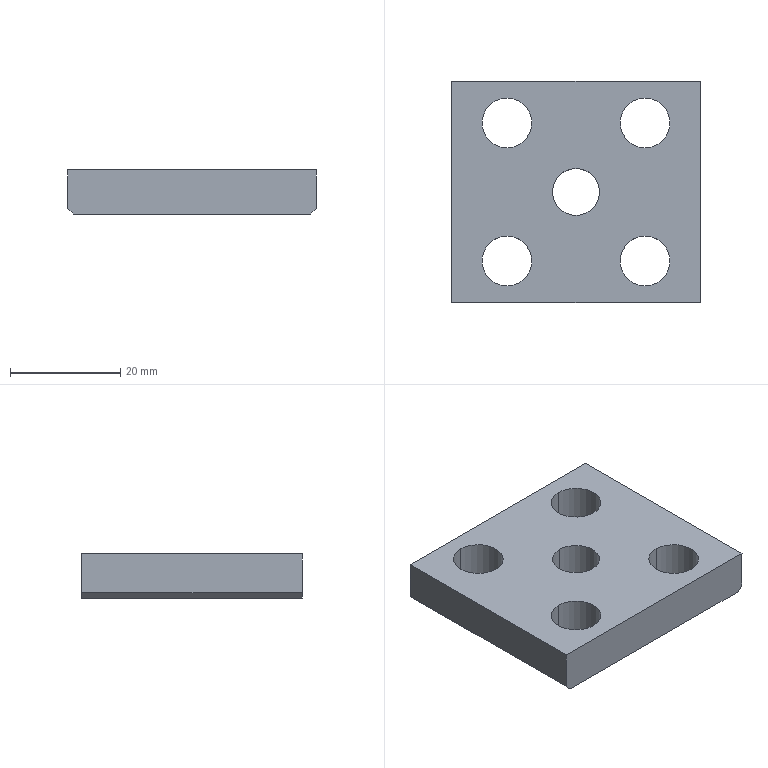Component | SolidWorks | Frame-1_PressurePlate-1 | 1 solid | 18 faces | box 45 x 40 x 8 mm | volume 11870 mm3 | cylinder 10 | plane 8 | commonest cylinder face diameters 9 x8 8.5 x2 | material Plain Carbon Steel
STEP:
#1=CARTESIAN_POINT('',(-171.122,344.501,294.147));
#2=VERTEX_POINT('',#1);
#3=CARTESIAN_POINT('',(-171.122,344.835,294.147));
#4=VERTEX_POINT('',#3);
#5=CARTESIAN_POINT('',(-171.122,344.668,294.147));
#6=DIRECTION('',(-0.,0.,-1.));
#7=DIRECTION('',(0.,1.,0.));
#8=AXIS2_PLACEMENT_3D('',#5,#6,#7);
#9=CIRCLE('',#8,0.1673);
#10=EDGE_CURVE('',#2,#4,#9,.T.);
#11=ORIENTED_EDGE('',*,*,#10,.F.);
#12=CARTESIAN_POINT('',(-171.122,344.501,293.832));
#13=VERTEX_POINT('',#12);
#14=CARTESIAN_POINT('',(-171.122,344.501,293.832));
#15=DIRECTION('',(-0.,0.,-1.));
#16=VECTOR('',#15,39.37);
#17=LINE('',#14,#16);
#18=EDGE_CURVE('',#2,#13,#17,.T.);
#19=ORIENTED_EDGE('',*,*,#18,.T.);
#20=CARTESIAN_POINT('',(-171.122,344.835,293.832));
#21=VERTEX_POINT('',#20);
#22=CARTESIAN_POINT('',(-171.122,344.668,293.832));
#23=DIRECTION('',(-0.,0.,-1.));
#24=DIRECTION('',(0.,1.,0.));
#25=AXIS2_PLACEMENT_3D('',#22,#23,#24);
#26=CIRCLE('',#25,0.1673);
#27=EDGE_CURVE('',#13,#21,#26,.T.);
#28=ORIENTED_EDGE('',*,*,#27,.T.);
#29=CARTESIAN_POINT('',(-171.122,344.835,293.832));
#30=DIRECTION('',(-0.,0.,-1.));
#31=VECTOR('',#30,39.37);
#32=LINE('',#29,#31);
#33=EDGE_CURVE('',#4,#21,#32,.T.);
#34=ORIENTED_EDGE('',*,*,#33,.F.);
#35=EDGE_LOOP('',(#11,#19,#28,#34));
#36=FACE_OUTER_BOUND('',#35,.T.);
#37=CARTESIAN_POINT('',(-171.122,344.668,293.832));
#38=DIRECTION('',(-0.,0.,-1.));
#39=DIRECTION('',(0.,1.,0.));
#40=AXIS2_PLACEMENT_3D('',#37,#38,#39);
#41=CYLINDRICAL_SURFACE('',#40,0.1673);
#42=ADVANCED_FACE('',(#36),#41,.F.);
#43=CARTESIAN_POINT('',(-171.614,343.999,293.832));
#44=VERTEX_POINT('',#43);
#45=CARTESIAN_POINT('',(-171.614,344.353,293.832));
#46=VERTEX_POINT('',#45);
#47=CARTESIAN_POINT('',(-171.614,344.176,293.832));
#48=DIRECTION('',(-0.,0.,-1.));
#49=DIRECTION('',(0.,1.,0.));
#50=AXIS2_PLACEMENT_3D('',#47,#48,#49);
#51=CIRCLE('',#50,0.1772);
#52=EDGE_CURVE('',#44,#46,#51,.T.);
#53=ORIENTED_EDGE('',*,*,#52,.T.);
#54=CARTESIAN_POINT('',(-171.614,344.353,294.147));
#55=VERTEX_POINT('',#54);
#56=CARTESIAN_POINT('',(-171.614,344.353,293.832));
#57=DIRECTION('',(0.,-0.,1.));
#58=VECTOR('',#57,39.37);
#59=LINE('',#56,#58);
#60=EDGE_CURVE('',#46,#55,#59,.T.);
#61=ORIENTED_EDGE('',*,*,#60,.T.);
#62=CARTESIAN_POINT('',(-171.614,343.999,294.147));
#63=VERTEX_POINT('',#62);
#64=CARTESIAN_POINT('',(-171.614,344.176,294.147));
#65=DIRECTION('',(-0.,0.,-1.));
#66=DIRECTION('',(0.,1.,0.));
#67=AXIS2_PLACEMENT_3D('',#64,#65,#66);
#68=CIRCLE('',#67,0.1772);
#69=EDGE_CURVE('',#63,#55,#68,.T.);
#70=ORIENTED_EDGE('',*,*,#69,.F.);
#71=CARTESIAN_POINT('',(-171.614,343.999,293.832));
#72=DIRECTION('',(0.,-0.,1.));
#73=VECTOR('',#72,39.37);
#74=LINE('',#71,#73);
#75=EDGE_CURVE('',#44,#63,#74,.T.);
#76=ORIENTED_EDGE('',*,*,#75,.F.);
#77=EDGE_LOOP('',(#53,#61,#70,#76));
#78=FACE_OUTER_BOUND('',#77,.T.);
#79=CARTESIAN_POINT('',(-171.614,344.176,293.832));
#80=DIRECTION('',(0.,-0.,1.));
#81=DIRECTION('',(-0.,-1.,0.));
#82=AXIS2_PLACEMENT_3D('',#79,#80,#81);
#83=CYLINDRICAL_SURFACE('',#82,0.1772);
#84=ADVANCED_FACE('',(#78),#83,.F.);
#85=CARTESIAN_POINT('',(-171.614,344.983,293.832));
#86=VERTEX_POINT('',#85);
#87=CARTESIAN_POINT('',(-171.614,345.337,293.832));
#88=VERTEX_POINT('',#87);
#89=CARTESIAN_POINT('',(-171.614,345.16,293.832));
#90=DIRECTION('',(-0.,0.,-1.));
#91=DIRECTION('',(0.,1.,0.));
#92=AXIS2_PLACEMENT_3D('',#89,#90,#91);
#93=CIRCLE('',#92,0.1772);
#94=EDGE_CURVE('',#86,#88,#93,.T.);
#95=ORIENTED_EDGE('',*,*,#94,.T.);
#96=CARTESIAN_POINT('',(-171.614,345.337,294.147));
#97=VERTEX_POINT('',#96);
#98=CARTESIAN_POINT('',(-171.614,345.337,293.832));
#99=DIRECTION('',(0.,-0.,1.));
#100=VECTOR('',#99,39.37);
#101=LINE('',#98,#100);
#102=EDGE_CURVE('',#88,#97,#101,.T.);
#103=ORIENTED_EDGE('',*,*,#102,.T.);
#104=CARTESIAN_POINT('',(-171.614,344.983,294.147));
#105=VERTEX_POINT('',#104);
#106=CARTESIAN_POINT('',(-171.614,345.16,294.147));
#107=DIRECTION('',(-0.,0.,-1.));
#108=DIRECTION('',(0.,1.,0.));
#109=AXIS2_PLACEMENT_3D('',#106,#107,#108);
#110=CIRCLE('',#109,0.1772);
#111=EDGE_CURVE('',#105,#97,#110,.T.);
#112=ORIENTED_EDGE('',*,*,#111,.F.);
#113=CARTESIAN_POINT('',(-171.614,344.983,293.832));
#114=DIRECTION('',(0.,-0.,1.));
#115=VECTOR('',#114,39.37);
#116=LINE('',#113,#115);
#117=EDGE_CURVE('',#86,#105,#116,.T.);
#118=ORIENTED_EDGE('',*,*,#117,.F.);
#119=EDGE_LOOP('',(#95,#103,#112,#118));
#120=FACE_OUTER_BOUND('',#119,.T.);
#121=CARTESIAN_POINT('',(-171.614,345.16,293.832));
#122=DIRECTION('',(0.,-0.,1.));
#123=DIRECTION('',(-0.,-1.,0.));
#124=AXIS2_PLACEMENT_3D('',#121,#122,#123);
#125=CYLINDRICAL_SURFACE('',#124,0.1772);
#126=ADVANCED_FACE('',(#120),#125,.F.);
#127=CARTESIAN_POINT('',(-170.63,343.999,293.832));
#128=VERTEX_POINT('',#127);
#129=CARTESIAN_POINT('',(-170.63,344.353,293.832));
#130=VERTEX_POINT('',#129);
#131=CARTESIAN_POINT('',(-170.63,344.176,293.832));
#132=DIRECTION('',(-0.,0.,-1.));
#133=DIRECTION('',(0.,1.,0.));
#134=AXIS2_PLACEMENT_3D('',#131,#132,#133);
#135=CIRCLE('',#134,0.1772);
#136=EDGE_CURVE('',#128,#130,#135,.T.);
#137=ORIENTED_EDGE('',*,*,#136,.T.);
#138=CARTESIAN_POINT('',(-170.63,344.353,294.147));
#139=VERTEX_POINT('',#138);
#140=CARTESIAN_POINT('',(-170.63,344.353,293.832));
#141=DIRECTION('',(0.,-0.,1.));
#142=VECTOR('',#141,39.37);
#143=LINE('',#140,#142);
#144=EDGE_CURVE('',#130,#139,#143,.T.);
#145=ORIENTED_EDGE('',*,*,#144,.T.);
#146=CARTESIAN_POINT('',(-170.63,343.999,294.147));
#147=VERTEX_POINT('',#146);
#148=CARTESIAN_POINT('',(-170.63,344.176,294.147));
#149=DIRECTION('',(-0.,0.,-1.));
#150=DIRECTION('',(0.,1.,0.));
#151=AXIS2_PLACEMENT_3D('',#148,#149,#150);
#152=CIRCLE('',#151,0.1772);
#153=EDGE_CURVE('',#147,#139,#152,.T.);
#154=ORIENTED_EDGE('',*,*,#153,.F.);
#155=CARTESIAN_POINT('',(-170.63,343.999,293.832));
#156=DIRECTION('',(0.,-0.,1.));
#157=VECTOR('',#156,39.37);
#158=LINE('',#155,#157);
#159=EDGE_CURVE('',#128,#147,#158,.T.);
#160=ORIENTED_EDGE('',*,*,#159,.F.);
#161=EDGE_LOOP('',(#137,#145,#154,#160));
#162=FACE_OUTER_BOUND('',#161,.T.);
#163=CARTESIAN_POINT('',(-170.63,344.176,293.832));
#164=DIRECTION('',(0.,-0.,1.));
#165=DIRECTION('',(-0.,-1.,0.));
#166=AXIS2_PLACEMENT_3D('',#163,#164,#165);
#167=CYLINDRICAL_SURFACE('',#166,0.1772);
#168=ADVANCED_FACE('',(#162),#167,.F.);
#169=CARTESIAN_POINT('',(-170.63,344.983,293.832));
#170=VERTEX_POINT('',#169);
#171=CARTESIAN_POINT('',(-170.63,345.337,293.832));
#172=VERTEX_POINT('',#171);
#173=CARTESIAN_POINT('',(-170.63,345.16,293.832));
#174=DIRECTION('',(-0.,0.,-1.));
#175=DIRECTION('',(0.,1.,0.));
#176=AXIS2_PLACEMENT_3D('',#173,#174,#175);
#177=CIRCLE('',#176,0.1772);
#178=EDGE_CURVE('',#170,#172,#177,.T.);
#179=ORIENTED_EDGE('',*,*,#178,.T.);
#180=CARTESIAN_POINT('',(-170.63,345.337,294.147));
#181=VERTEX_POINT('',#180);
#182=CARTESIAN_POINT('',(-170.63,345.337,293.832));
#183=DIRECTION('',(0.,-0.,1.));
#184=VECTOR('',#183,39.37);
#185=LINE('',#182,#184);
#186=EDGE_CURVE('',#172,#181,#185,.T.);
#187=ORIENTED_EDGE('',*,*,#186,.T.);
#188=CARTESIAN_POINT('',(-170.63,344.983,294.147));
#189=VERTEX_POINT('',#188);
#190=CARTESIAN_POINT('',(-170.63,345.16,294.147));
#191=DIRECTION('',(-0.,0.,-1.));
#192=DIRECTION('',(0.,1.,0.));
#193=AXIS2_PLACEMENT_3D('',#190,#191,#192);
#194=CIRCLE('',#193,0.1772);
#195=EDGE_CURVE('',#189,#181,#194,.T.);
#196=ORIENTED_EDGE('',*,*,#195,.F.);
#197=CARTESIAN_POINT('',(-170.63,344.983,293.832));
#198=DIRECTION('',(0.,-0.,1.));
#199=VECTOR('',#198,39.37);
#200=LINE('',#197,#199);
#201=EDGE_CURVE('',#170,#189,#200,.T.);
#202=ORIENTED_EDGE('',*,*,#201,.F.);
#203=EDGE_LOOP('',(#179,#187,#196,#202));
#204=FACE_OUTER_BOUND('',#203,.T.);
#205=CARTESIAN_POINT('',(-170.63,345.16,293.832));
#206=DIRECTION('',(0.,-0.,1.));
#207=DIRECTION('',(-0.,-1.,0.));
#208=AXIS2_PLACEMENT_3D('',#205,#206,#207);
#209=CYLINDRICAL_SURFACE('',#208,0.1772);
#210=ADVANCED_FACE('',(#204),#209,.F.);
#211=CARTESIAN_POINT('',(-171.122,344.668,293.832));
#212=DIRECTION('',(-0.,0.,-1.));
#213=DIRECTION('',(0.,1.,0.));
#214=AXIS2_PLACEMENT_3D('',#211,#212,#213);
#215=CIRCLE('',#214,0.1673);
#216=EDGE_CURVE('',#21,#13,#215,.T.);
#217=ORIENTED_EDGE('',*,*,#216,.F.);
#218=ORIENTED_EDGE('',*,*,#27,.F.);
#219=EDGE_LOOP('',(#217,#218));
#220=FACE_BOUND('',#219,.T.);
#221=CARTESIAN_POINT('',(-170.276,343.88,293.832));
#222=VERTEX_POINT('',#221);
#223=CARTESIAN_POINT('',(-171.969,343.88,293.832));
#224=VERTEX_POINT('',#223);
#225=CARTESIAN_POINT('',(-172.008,343.88,293.832));
#226=DIRECTION('',(-1.,0.,0.));
#227=VECTOR('',#226,39.37);
#228=LINE('',#225,#227);
#229=EDGE_CURVE('',#222,#224,#228,.T.);
#230=ORIENTED_EDGE('',*,*,#229,.T.);
#231=CARTESIAN_POINT('',(-171.969,345.455,293.832));
#232=VERTEX_POINT('',#231);
#233=CARTESIAN_POINT('',(-171.969,343.88,293.832));
#234=DIRECTION('',(0.,1.,0.));
#235=VECTOR('',#234,39.37);
#236=LINE('',#233,#235);
#237=EDGE_CURVE('',#224,#232,#236,.T.);
#238=ORIENTED_EDGE('',*,*,#237,.T.);
#239=CARTESIAN_POINT('',(-170.276,345.455,293.832));
#240=VERTEX_POINT('',#239);
#241=CARTESIAN_POINT('',(-172.008,345.455,293.832));
#242=DIRECTION('',(1.,-0.,-0.));
#243=VECTOR('',#242,39.37);
#244=LINE('',#241,#243);
#245=EDGE_CURVE('',#232,#240,#244,.T.);
#246=ORIENTED_EDGE('',*,*,#245,.T.);
#247=CARTESIAN_POINT('',(-170.276,343.88,293.832));
#248=DIRECTION('',(-0.,-1.,-0.));
#249=VECTOR('',#248,39.37);
#250=LINE('',#247,#249);
#251=EDGE_CURVE('',#240,#222,#250,.T.);
#252=ORIENTED_EDGE('',*,*,#251,.T.);
#253=EDGE_LOOP('',(#230,#238,#246,#252));
#254=FACE_OUTER_BOUND('',#253,.T.);
#255=ORIENTED_EDGE('',*,*,#178,.F.);
#256=CARTESIAN_POINT('',(-170.63,345.16,293.832));
#257=DIRECTION('',(-0.,0.,-1.));
#258=DIRECTION('',(0.,1.,0.));
#259=AXIS2_PLACEMENT_3D('',#256,#257,#258);
#260=CIRCLE('',#259,0.1772);
#261=EDGE_CURVE('',#172,#170,#260,.T.);
#262=ORIENTED_EDGE('',*,*,#261,.F.);
#263=EDGE_LOOP('',(#255,#262));
#264=FACE_BOUND('',#263,.T.);
#265=ORIENTED_EDGE('',*,*,#136,.F.);
#266=CARTESIAN_POINT('',(-170.63,344.176,293.832));
#267=DIRECTION('',(-0.,0.,-1.));
#268=DIRECTION('',(0.,1.,0.));
#269=AXIS2_PLACEMENT_3D('',#266,#267,#268);
#270=CIRCLE('',#269,0.1772);
#271=EDGE_CURVE('',#130,#128,#270,.T.);
#272=ORIENTED_EDGE('',*,*,#271,.F.);
#273=EDGE_LOOP('',(#265,#272));
#274=FACE_BOUND('',#273,.T.);
#275=ORIENTED_EDGE('',*,*,#94,.F.);
#276=CARTESIAN_POINT('',(-171.614,345.16,293.832));
#277=DIRECTION('',(-0.,0.,-1.));
#278=DIRECTION('',(0.,1.,0.));
#279=AXIS2_PLACEMENT_3D('',#276,#277,#278);
#280=CIRCLE('',#279,0.1772);
#281=EDGE_CURVE('',#88,#86,#280,.T.);
#282=ORIENTED_EDGE('',*,*,#281,.F.);
#283=EDGE_LOOP('',(#275,#282));
#284=FACE_BOUND('',#283,.T.);
#285=ORIENTED_EDGE('',*,*,#52,.F.);
#286=CARTESIAN_POINT('',(-171.614,344.176,293.832));
#287=DIRECTION('',(-0.,0.,-1.));
#288=DIRECTION('',(0.,1.,0.));
#289=AXIS2_PLACEMENT_3D('',#286,#287,#288);
#290=CIRCLE('',#289,0.1772);
#291=EDGE_CURVE('',#46,#44,#290,.T.);
#292=ORIENTED_EDGE('',*,*,#291,.F.);
#293=EDGE_LOOP('',(#285,#292));
#294=FACE_BOUND('',#293,.T.);
#295=CARTESIAN_POINT('',(-170.236,343.88,293.832));
#296=DIRECTION('',(0.,-0.,1.));
#297=DIRECTION('',(-0.,-1.,-0.));
#298=AXIS2_PLACEMENT_3D('',#295,#296,#297);
#299=PLANE('',#298);
#300=ADVANCED_FACE('',(#220,#254,#264,#274,#284,#294),#299,.F.);
#301=CARTESIAN_POINT('',(-171.122,344.668,294.147));
#302=DIRECTION('',(-0.,0.,-1.));
#303=DIRECTION('',(0.,1.,0.));
#304=AXIS2_PLACEMENT_3D('',#301,#302,#303);
#305=CIRCLE('',#304,0.1673);
#306=EDGE_CURVE('',#4,#2,#305,.T.);
#307=ORIENTED_EDGE('',*,*,#306,.T.);
#308=ORIENTED_EDGE('',*,*,#10,.T.);
#309=EDGE_LOOP('',(#307,#308));
#310=FACE_BOUND('',#309,.T.);
#311=ORIENTED_EDGE('',*,*,#111,.T.);
#312=CARTESIAN_POINT('',(-171.614,345.16,294.147));
#313=DIRECTION('',(-0.,0.,-1.));
#314=DIRECTION('',(0.,1.,0.));
#315=AXIS2_PLACEMENT_3D('',#312,#313,#314);
#316=CIRCLE('',#315,0.1772);
#317=EDGE_CURVE('',#97,#105,#316,.T.);
#318=ORIENTED_EDGE('',*,*,#317,.T.);
#319=EDGE_LOOP('',(#311,#318));
#320=FACE_BOUND('',#319,.T.);
#321=ORIENTED_EDGE('',*,*,#195,.T.);
#322=CARTESIAN_POINT('',(-170.63,345.16,294.147));
#323=DIRECTION('',(-0.,0.,-1.));
#324=DIRECTION('',(0.,1.,0.));
#325=AXIS2_PLACEMENT_3D('',#322,#323,#324);
#326=CIRCLE('',#325,0.1772);
#327=EDGE_CURVE('',#181,#189,#326,.T.);
#328=ORIENTED_EDGE('',*,*,#327,.T.);
#329=EDGE_LOOP('',(#321,#328));
#330=FACE_BOUND('',#329,.T.);
#331=CARTESIAN_POINT('',(-170.236,343.88,294.147));
#332=VERTEX_POINT('',#331);
#333=CARTESIAN_POINT('',(-172.008,343.88,294.147));
#334=VERTEX_POINT('',#333);
#335=CARTESIAN_POINT('',(-172.008,343.88,294.147));
#336=DIRECTION('',(-1.,0.,0.));
#337=VECTOR('',#336,39.37);
#338=LINE('',#335,#337);
#339=EDGE_CURVE('',#332,#334,#338,.T.);
#340=ORIENTED_EDGE('',*,*,#339,.F.);
#341=CARTESIAN_POINT('',(-170.236,345.455,294.147));
#342=VERTEX_POINT('',#341);
#343=CARTESIAN_POINT('',(-170.236,343.88,294.147));
#344=DIRECTION('',(-0.,-1.,-0.));
#345=VECTOR('',#344,39.37);
#346=LINE('',#343,#345);
#347=EDGE_CURVE('',#342,#332,#346,.T.);
#348=ORIENTED_EDGE('',*,*,#347,.F.);
#349=CARTESIAN_POINT('',(-172.008,345.455,294.147));
#350=VERTEX_POINT('',#349);
#351=CARTESIAN_POINT('',(-172.008,345.455,294.147));
#352=DIRECTION('',(1.,-0.,-0.));
#353=VECTOR('',#352,39.37);
#354=LINE('',#351,#353);
#355=EDGE_CURVE('',#350,#342,#354,.T.);
#356=ORIENTED_EDGE('',*,*,#355,.F.);
#357=CARTESIAN_POINT('',(-172.008,343.88,294.147));
#358=DIRECTION('',(0.,1.,0.));
#359=VECTOR('',#358,39.37);
#360=LINE('',#357,#359);
#361=EDGE_CURVE('',#334,#350,#360,.T.);
#362=ORIENTED_EDGE('',*,*,#361,.F.);
#363=EDGE_LOOP('',(#340,#348,#356,#362));
#364=FACE_OUTER_BOUND('',#363,.T.);
#365=ORIENTED_EDGE('',*,*,#153,.T.);
#366=CARTESIAN_POINT('',(-170.63,344.176,294.147));
#367=DIRECTION('',(-0.,0.,-1.));
#368=DIRECTION('',(0.,1.,0.));
#369=AXIS2_PLACEMENT_3D('',#366,#367,#368);
#370=CIRCLE('',#369,0.1772);
#371=EDGE_CURVE('',#139,#147,#370,.T.);
#372=ORIENTED_EDGE('',*,*,#371,.T.);
#373=EDGE_LOOP('',(#365,#372));
#374=FACE_BOUND('',#373,.T.);
#375=ORIENTED_EDGE('',*,*,#69,.T.);
#376=CARTESIAN_POINT('',(-171.614,344.176,294.147));
#377=DIRECTION('',(-0.,0.,-1.));
#378=DIRECTION('',(0.,1.,0.));
#379=AXIS2_PLACEMENT_3D('',#376,#377,#378);
#380=CIRCLE('',#379,0.1772);
#381=EDGE_CURVE('',#55,#63,#380,.T.);
#382=ORIENTED_EDGE('',*,*,#381,.T.);
#383=EDGE_LOOP('',(#375,#382));
#384=FACE_BOUND('',#383,.T.);
#385=CARTESIAN_POINT('',(-170.236,343.88,294.147));
#386=DIRECTION('',(0.,-0.,1.));
#387=DIRECTION('',(-0.,-1.,-0.));
#388=AXIS2_PLACEMENT_3D('',#385,#386,#387);
#389=PLANE('',#388);
#390=ADVANCED_FACE('',(#310,#320,#330,#364,#374,#384),#389,.T.);
#391=CARTESIAN_POINT('',(-172.008,343.88,293.872));
#392=VERTEX_POINT('',#391);
#393=CARTESIAN_POINT('',(-172.008,343.88,293.832));
#394=DIRECTION('',(0.,-0.,1.));
#395=VECTOR('',#394,39.37);
#396=LINE('',#393,#395);
#397=EDGE_CURVE('',#392,#334,#396,.T.);
#398=ORIENTED_EDGE('',*,*,#397,.F.);
#399=CARTESIAN_POINT('',(-171.969,343.88,293.832));
#400=DIRECTION('',(0.7071,-0.,-0.7071));
#401=VECTOR('',#400,39.37);
#402=LINE('',#399,#401);
#403=EDGE_CURVE('',#392,#224,#402,.T.);
#404=ORIENTED_EDGE('',*,*,#403,.T.);
#405=ORIENTED_EDGE('',*,*,#229,.F.);
#406=CARTESIAN_POINT('',(-170.236,343.88,293.872));
#407=VERTEX_POINT('',#406);
#408=CARTESIAN_POINT('',(-170.276,343.88,293.832));
#409=DIRECTION('',(0.7071,-0.,0.7071));
#410=VECTOR('',#409,39.37);
#411=LINE('',#408,#410);
#412=EDGE_CURVE('',#222,#407,#411,.T.);
#413=ORIENTED_EDGE('',*,*,#412,.T.);
#414=CARTESIAN_POINT('',(-170.236,343.88,293.832));
#415=DIRECTION('',(0.,-0.,1.));
#416=VECTOR('',#415,39.37);
#417=LINE('',#414,#416);
#418=EDGE_CURVE('',#407,#332,#417,.T.);
#419=ORIENTED_EDGE('',*,*,#418,.T.);
#420=ORIENTED_EDGE('',*,*,#339,.T.);
#421=EDGE_LOOP('',(#398,#404,#405,#413,#419,#420));
#422=FACE_OUTER_BOUND('',#421,.T.);
#423=CARTESIAN_POINT('',(-172.008,343.88,293.832));
#424=DIRECTION('',(0.,1.,0.));
#425=DIRECTION('',(0.,-0.,1.));
#426=AXIS2_PLACEMENT_3D('',#423,#424,#425);
#427=PLANE('',#426);
#428=ADVANCED_FACE('',(#422),#427,.F.);
#429=CARTESIAN_POINT('',(-172.008,345.455,293.872));
#430=VERTEX_POINT('',#429);
#431=CARTESIAN_POINT('',(-172.008,345.455,293.832));
#432=DIRECTION('',(0.,-0.,1.));
#433=VECTOR('',#432,39.37);
#434=LINE('',#431,#433);
#435=EDGE_CURVE('',#430,#350,#434,.T.);
#436=ORIENTED_EDGE('',*,*,#435,.F.);
#437=CARTESIAN_POINT('',(-172.008,343.88,293.872));
#438=DIRECTION('',(-0.,-1.,-0.));
#439=VECTOR('',#438,39.37);
#440=LINE('',#437,#439);
#441=EDGE_CURVE('',#430,#392,#440,.T.);
#442=ORIENTED_EDGE('',*,*,#441,.T.);
#443=ORIENTED_EDGE('',*,*,#397,.T.);
#444=ORIENTED_EDGE('',*,*,#361,.T.);
#445=EDGE_LOOP('',(#436,#442,#443,#444));
#446=FACE_OUTER_BOUND('',#445,.T.);
#447=CARTESIAN_POINT('',(-172.008,343.88,293.832));
#448=DIRECTION('',(1.,-0.,-0.));
#449=DIRECTION('',(-0.,0.,-1.));
#450=AXIS2_PLACEMENT_3D('',#447,#448,#449);
#451=PLANE('',#450);
#452=ADVANCED_FACE('',(#446),#451,.F.);
#453=ORIENTED_EDGE('',*,*,#245,.F.);
#454=CARTESIAN_POINT('',(-171.969,345.455,293.832));
#455=DIRECTION('',(-0.7071,0.,0.7071));
#456=VECTOR('',#455,39.37);
#457=LINE('',#454,#456);
#458=EDGE_CURVE('',#232,#430,#457,.T.);
#459=ORIENTED_EDGE('',*,*,#458,.T.);
#460=ORIENTED_EDGE('',*,*,#435,.T.);
#461=ORIENTED_EDGE('',*,*,#355,.T.);
#462=CARTESIAN_POINT('',(-170.236,345.455,293.872));
#463=VERTEX_POINT('',#462);
#464=CARTESIAN_POINT('',(-170.236,345.455,293.832));
#465=DIRECTION('',(0.,-0.,1.));
#466=VECTOR('',#465,39.37);
#467=LINE('',#464,#466);
#468=EDGE_CURVE('',#463,#342,#467,.T.);
#469=ORIENTED_EDGE('',*,*,#468,.F.);
#470=CARTESIAN_POINT('',(-170.276,345.455,293.832));
#471=DIRECTION('',(-0.7071,0.,-0.7071));
#472=VECTOR('',#471,39.37);
#473=LINE('',#470,#472);
#474=EDGE_CURVE('',#463,#240,#473,.T.);
#475=ORIENTED_EDGE('',*,*,#474,.T.);
#476=EDGE_LOOP('',(#453,#459,#460,#461,#469,#475));
#477=FACE_OUTER_BOUND('',#476,.T.);
#478=CARTESIAN_POINT('',(-172.008,345.455,293.832));
#479=DIRECTION('',(-0.,-1.,-0.));
#480=DIRECTION('',(-0.,0.,-1.));
#481=AXIS2_PLACEMENT_3D('',#478,#479,#480);
#482=PLANE('',#481);
#483=ADVANCED_FACE('',(#477),#482,.F.);
#484=ORIENTED_EDGE('',*,*,#418,.F.);
#485=CARTESIAN_POINT('',(-170.236,343.88,293.872));
#486=DIRECTION('',(0.,1.,0.));
#487=VECTOR('',#486,39.37);
#488=LINE('',#485,#487);
#489=EDGE_CURVE('',#407,#463,#488,.T.);
#490=ORIENTED_EDGE('',*,*,#489,.T.);
#491=ORIENTED_EDGE('',*,*,#468,.T.);
#492=ORIENTED_EDGE('',*,*,#347,.T.);
#493=EDGE_LOOP('',(#484,#490,#491,#492));
#494=FACE_OUTER_BOUND('',#493,.T.);
#495=CARTESIAN_POINT('',(-170.236,343.88,293.832));
#496=DIRECTION('',(-1.,0.,0.));
#497=DIRECTION('',(0.,-0.,1.));
#498=AXIS2_PLACEMENT_3D('',#495,#496,#497);
#499=PLANE('',#498);
#500=ADVANCED_FACE('',(#494),#499,.F.);
#501=ORIENTED_EDGE('',*,*,#186,.F.);
#502=ORIENTED_EDGE('',*,*,#261,.T.);
#503=ORIENTED_EDGE('',*,*,#201,.T.);
#504=ORIENTED_EDGE('',*,*,#327,.F.);
#505=EDGE_LOOP('',(#501,#502,#503,#504));
#506=FACE_OUTER_BOUND('',#505,.T.);
#507=CARTESIAN_POINT('',(-170.63,345.16,293.832));
#508=DIRECTION('',(0.,-0.,1.));
#509=DIRECTION('',(-0.,-1.,0.));
#510=AXIS2_PLACEMENT_3D('',#507,#508,#509);
#511=CYLINDRICAL_SURFACE('',#510,0.1772);
#512=ADVANCED_FACE('',(#506),#511,.F.);
#513=ORIENTED_EDGE('',*,*,#144,.F.);
#514=ORIENTED_EDGE('',*,*,#271,.T.);
#515=ORIENTED_EDGE('',*,*,#159,.T.);
#516=ORIENTED_EDGE('',*,*,#371,.F.);
#517=EDGE_LOOP('',(#513,#514,#515,#516));
#518=FACE_OUTER_BOUND('',#517,.T.);
#519=CARTESIAN_POINT('',(-170.63,344.176,293.832));
#520=DIRECTION('',(0.,-0.,1.));
#521=DIRECTION('',(-0.,-1.,0.));
#522=AXIS2_PLACEMENT_3D('',#519,#520,#521);
#523=CYLINDRICAL_SURFACE('',#522,0.1772);
#524=ADVANCED_FACE('',(#518),#523,.F.);
#525=ORIENTED_EDGE('',*,*,#102,.F.);
#526=ORIENTED_EDGE('',*,*,#281,.T.);
#527=ORIENTED_EDGE('',*,*,#117,.T.);
#528=ORIENTED_EDGE('',*,*,#317,.F.);
#529=EDGE_LOOP('',(#525,#526,#527,#528));
#530=FACE_OUTER_BOUND('',#529,.T.);
#531=CARTESIAN_POINT('',(-171.614,345.16,293.832));
#532=DIRECTION('',(0.,-0.,1.));
#533=DIRECTION('',(-0.,-1.,0.));
#534=AXIS2_PLACEMENT_3D('',#531,#532,#533);
#535=CYLINDRICAL_SURFACE('',#534,0.1772);
#536=ADVANCED_FACE('',(#530),#535,.F.);
#537=ORIENTED_EDGE('',*,*,#60,.F.);
#538=ORIENTED_EDGE('',*,*,#291,.T.);
#539=ORIENTED_EDGE('',*,*,#75,.T.);
#540=ORIENTED_EDGE('',*,*,#381,.F.);
#541=EDGE_LOOP('',(#537,#538,#539,#540));
#542=FACE_OUTER_BOUND('',#541,.T.);
#543=CARTESIAN_POINT('',(-171.614,344.176,293.832));
#544=DIRECTION('',(0.,-0.,1.));
#545=DIRECTION('',(-0.,-1.,0.));
#546=AXIS2_PLACEMENT_3D('',#543,#544,#545);
#547=CYLINDRICAL_SURFACE('',#546,0.1772);
#548=ADVANCED_FACE('',(#542),#547,.F.);
#549=ORIENTED_EDGE('',*,*,#18,.F.);
#550=ORIENTED_EDGE('',*,*,#306,.F.);
#551=ORIENTED_EDGE('',*,*,#33,.T.);
#552=ORIENTED_EDGE('',*,*,#216,.T.);
#553=EDGE_LOOP('',(#549,#550,#551,#552));
#554=FACE_OUTER_BOUND('',#553,.T.);
#555=CARTESIAN_POINT('',(-171.122,344.668,293.832));
#556=DIRECTION('',(-0.,0.,-1.));
#557=DIRECTION('',(0.,1.,0.));
#558=AXIS2_PLACEMENT_3D('',#555,#556,#557);
#559=CYLINDRICAL_SURFACE('',#558,0.1673);
#560=ADVANCED_FACE('',(#554),#559,.F.);
#561=ORIENTED_EDGE('',*,*,#403,.F.);
#562=ORIENTED_EDGE('',*,*,#441,.F.);
#563=ORIENTED_EDGE('',*,*,#458,.F.);
#564=ORIENTED_EDGE('',*,*,#237,.F.);
#565=EDGE_LOOP('',(#561,#562,#563,#564));
#566=FACE_OUTER_BOUND('',#565,.T.);
#567=CARTESIAN_POINT('',(-171.969,343.88,293.832));
#568=DIRECTION('',(0.7071,-0.,0.7071));
#569=DIRECTION('',(0.,1.,0.));
#570=AXIS2_PLACEMENT_3D('',#567,#568,#569);
#571=PLANE('',#570);
#572=ADVANCED_FACE('',(#566),#571,.F.);
#573=ORIENTED_EDGE('',*,*,#474,.F.);
#574=ORIENTED_EDGE('',*,*,#489,.F.);
#575=ORIENTED_EDGE('',*,*,#412,.F.);
#576=ORIENTED_EDGE('',*,*,#251,.F.);
#577=EDGE_LOOP('',(#573,#574,#575,#576));
#578=FACE_OUTER_BOUND('',#577,.T.);
#579=CARTESIAN_POINT('',(-170.276,343.88,293.832));
#580=DIRECTION('',(-0.7071,0.,0.7071));
#581=DIRECTION('',(-0.,-1.,-0.));
#582=AXIS2_PLACEMENT_3D('',#579,#580,#581);
#583=PLANE('',#582);
#584=ADVANCED_FACE('',(#578),#583,.F.);
#585=CLOSED_SHELL('',(#42,#84,#126,#168,#210,#300,#390,#428,#452,#483,#500,#512,#524,#536,#548,#560,#572,#584));
#586=MANIFOLD_SOLID_BREP('',#585);
#587=CARTESIAN_POINT('',(0.,0.,0.));
#588=DIRECTION('',(0.,0.,1.));
#589=DIRECTION('',(1.,0.,0.));
#590=AXIS2_PLACEMENT_3D('',#587,#588,#589);
#591=(LENGTH_UNIT()NAMED_UNIT(*)SI_UNIT($,.METRE.));
#592=LENGTH_MEASURE_WITH_UNIT(LENGTH_MEASURE(0.0254),#591);
#593=DIMENSIONAL_EXPONENTS(1.,0.,0.,0.,0.,0.,0.);
#594=(CONVERSION_BASED_UNIT('',#592)LENGTH_UNIT()NAMED_UNIT(#593));
#595=UNCERTAINTY_MEASURE_WITH_UNIT(LENGTH_MEASURE(0.00001),#594,'','');
#596=(NAMED_UNIT(*)PLANE_ANGLE_UNIT()SI_UNIT($,.RADIAN.));
#597=(NAMED_UNIT(*)SI_UNIT($,.STERADIAN.)SOLID_ANGLE_UNIT());
#598=(GEOMETRIC_REPRESENTATION_CONTEXT(3)GLOBAL_UNCERTAINTY_ASSIGNED_CONTEXT((#595))GLOBAL_UNIT_ASSIGNED_CONTEXT((#594,#596,#597))REPRESENTATION_CONTEXT('',''));
#599=ADVANCED_BREP_SHAPE_REPRESENTATION('',(#586,#590),#598);
#600=COLOUR_RGB('',0.7922,0.8196,0.9333);
#601=FILL_AREA_STYLE_COLOUR('',#600);
#602=FILL_AREA_STYLE('',(#601));
#603=SURFACE_STYLE_FILL_AREA(#602);
#604=SURFACE_SIDE_STYLE('',(#603));
#605=SURFACE_STYLE_USAGE(.BOTH.,#604);
#606=PRESENTATION_STYLE_ASSIGNMENT((#605));
#607=STYLED_ITEM('',(#606),#586);
#608=PRESENTATION_LAYER_ASSIGNMENT('','',(#607));
#609=(LENGTH_UNIT()NAMED_UNIT(*)SI_UNIT($,.METRE.));
#610=LENGTH_MEASURE_WITH_UNIT(LENGTH_MEASURE(0.0254),#609);
#611=DIMENSIONAL_EXPONENTS(1.,0.,0.,0.,0.,0.,0.);
#612=(CONVERSION_BASED_UNIT('',#610)LENGTH_UNIT()NAMED_UNIT(#611));
#613=UNCERTAINTY_MEASURE_WITH_UNIT(LENGTH_MEASURE(0.00001),#612,'','');
#614=(NAMED_UNIT(*)PLANE_ANGLE_UNIT()SI_UNIT($,.RADIAN.));
#615=(NAMED_UNIT(*)SI_UNIT($,.STERADIAN.)SOLID_ANGLE_UNIT());
#616=(GEOMETRIC_REPRESENTATION_CONTEXT(3)GLOBAL_UNCERTAINTY_ASSIGNED_CONTEXT((#613))GLOBAL_UNIT_ASSIGNED_CONTEXT((#612,#614,#615))REPRESENTATION_CONTEXT('',''));
#617=MECHANICAL_DESIGN_GEOMETRIC_PRESENTATION_REPRESENTATION('',(#607),#616);